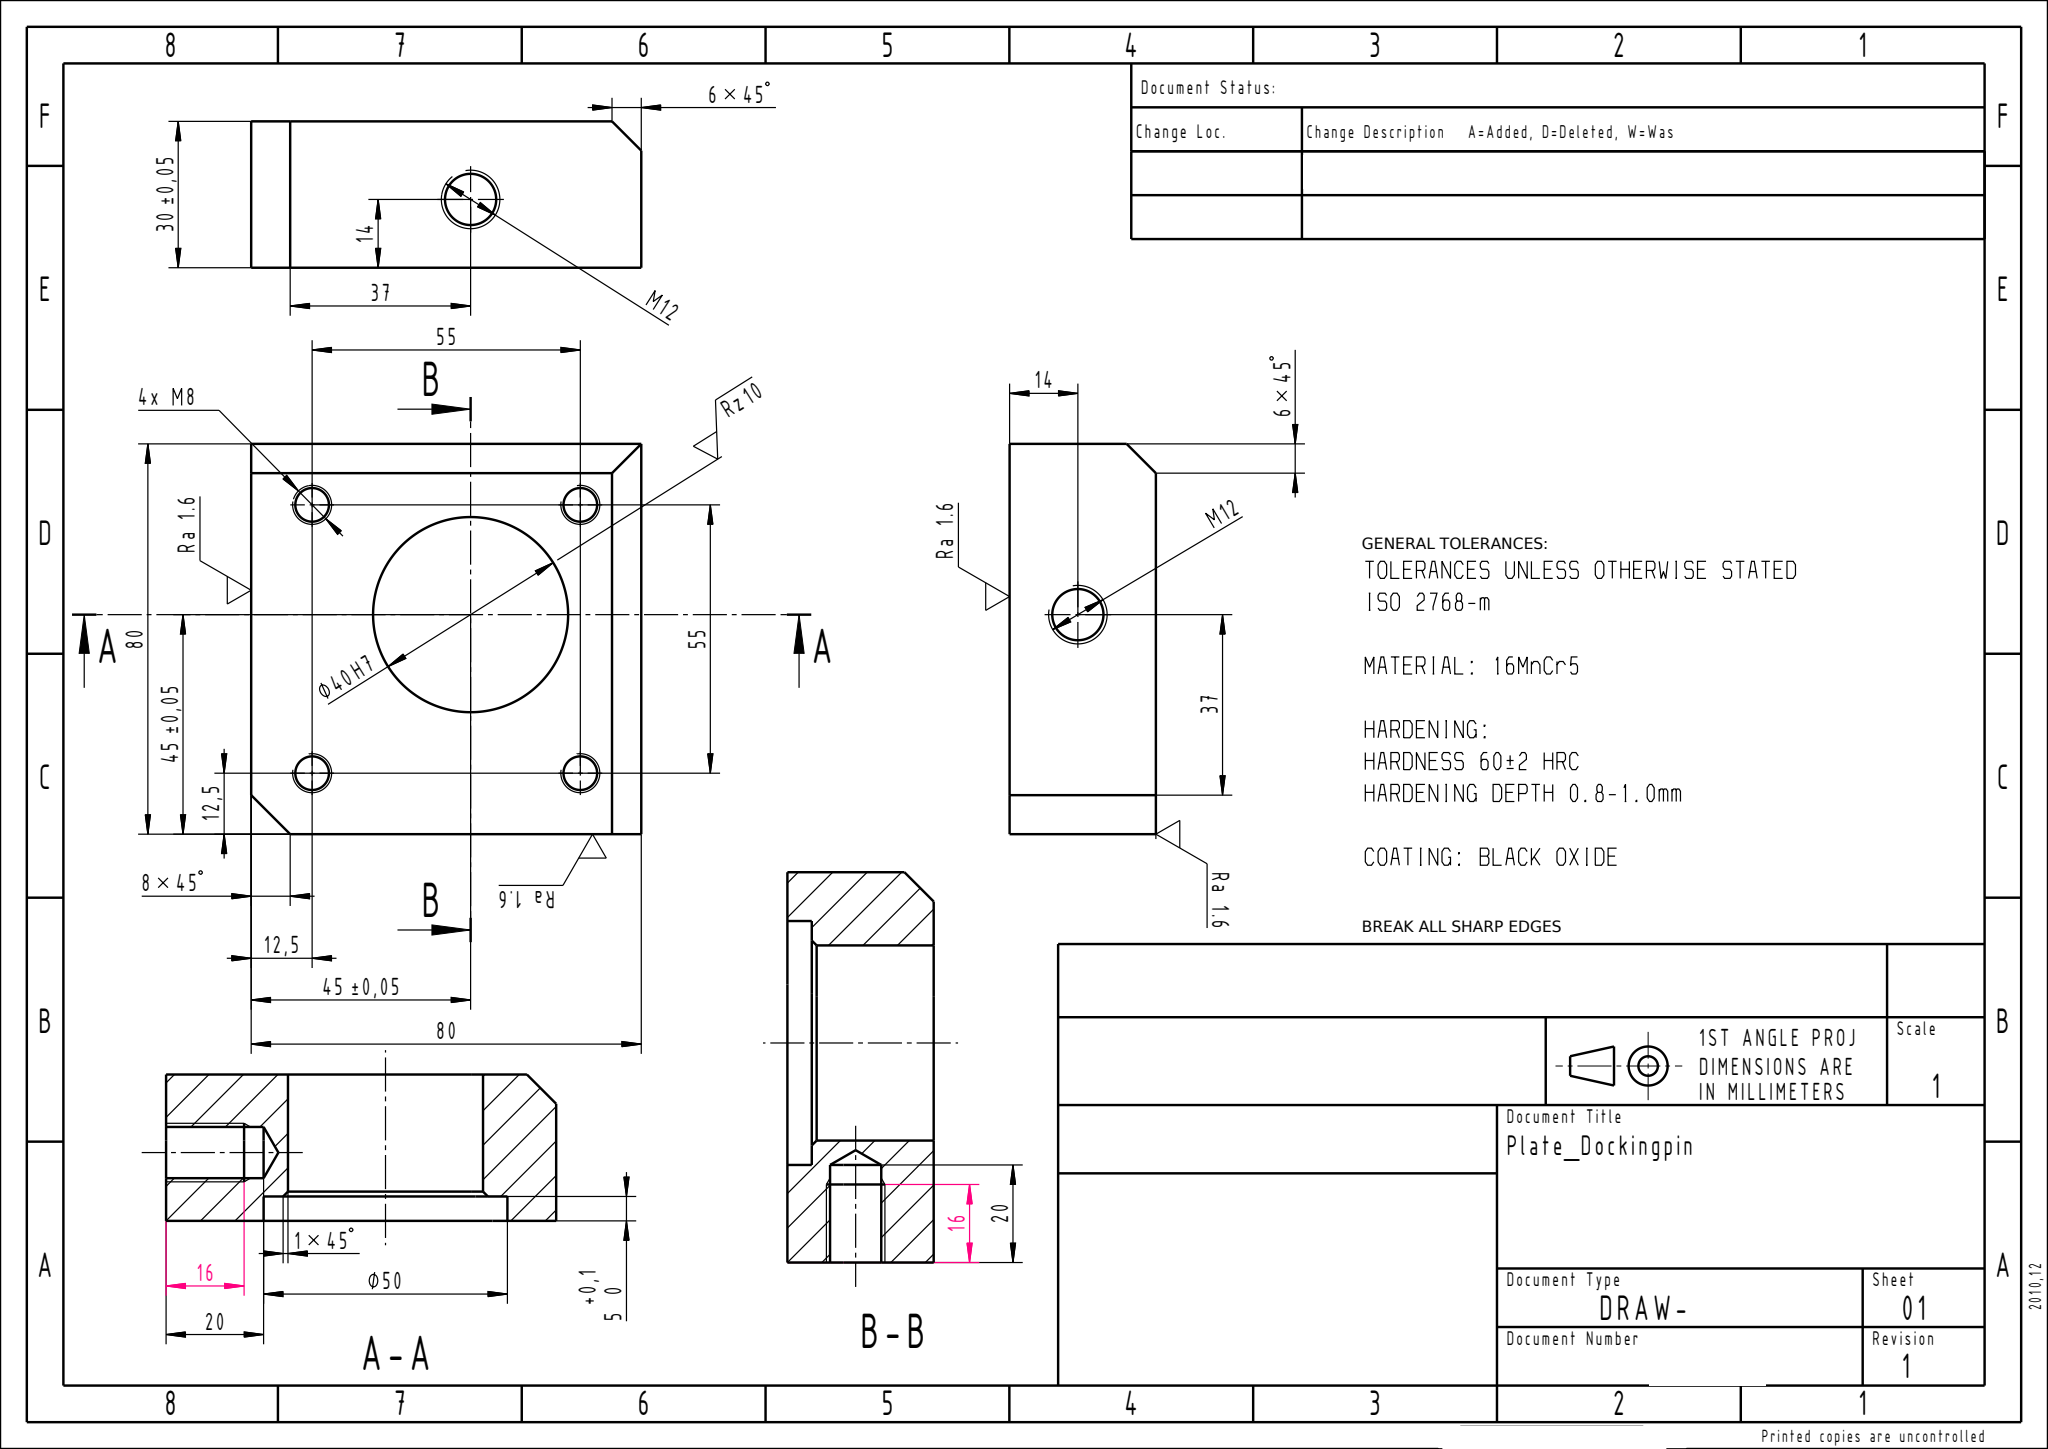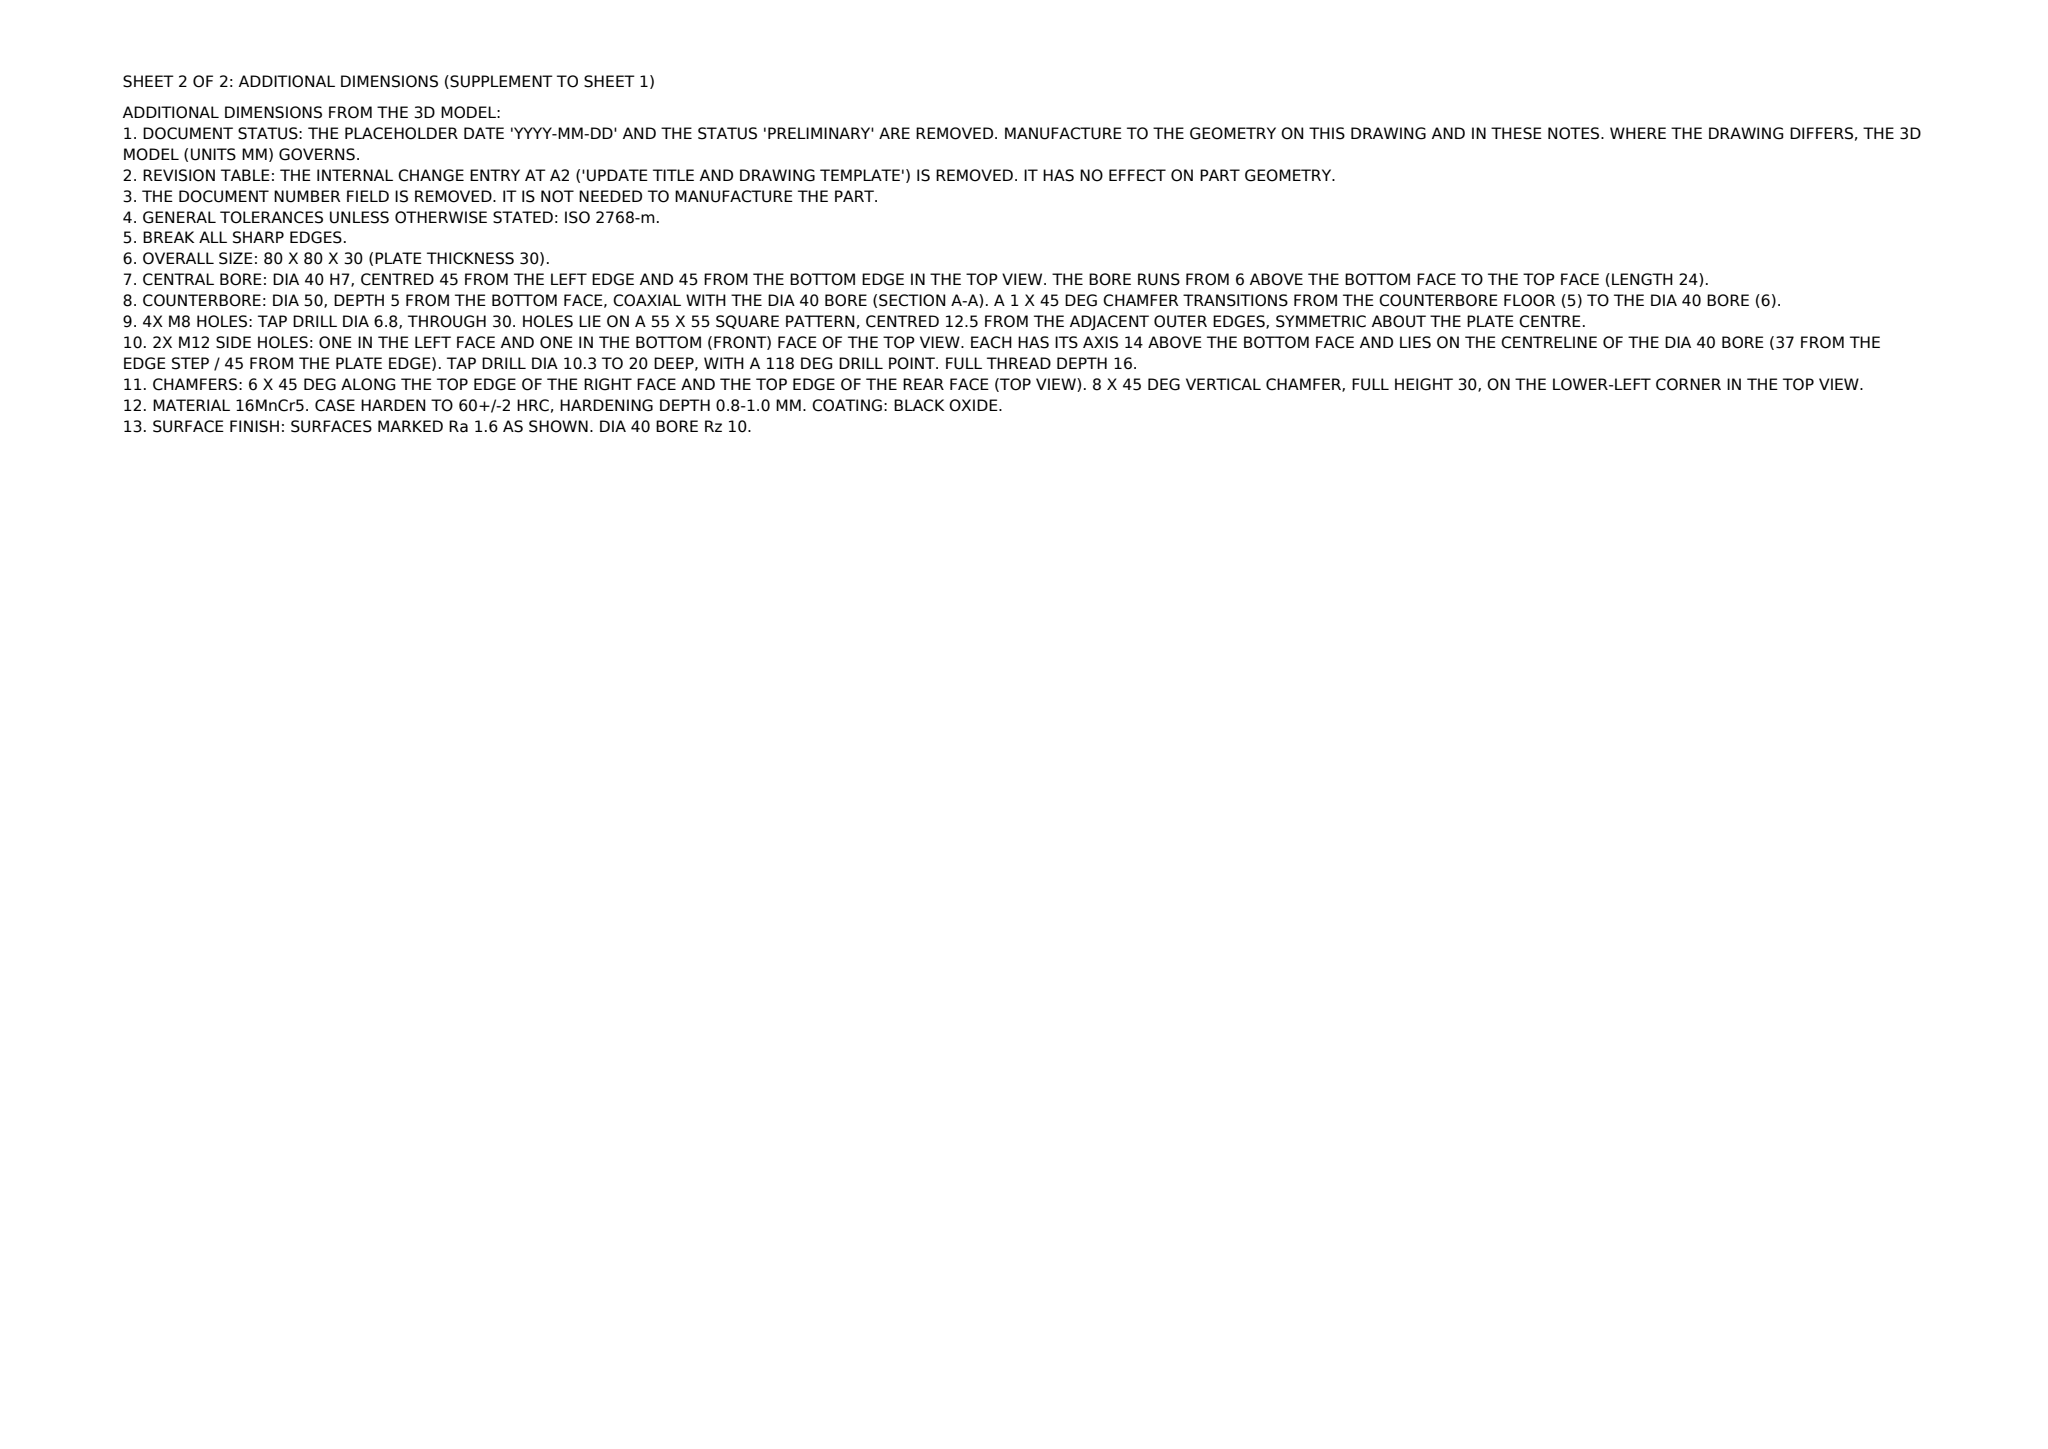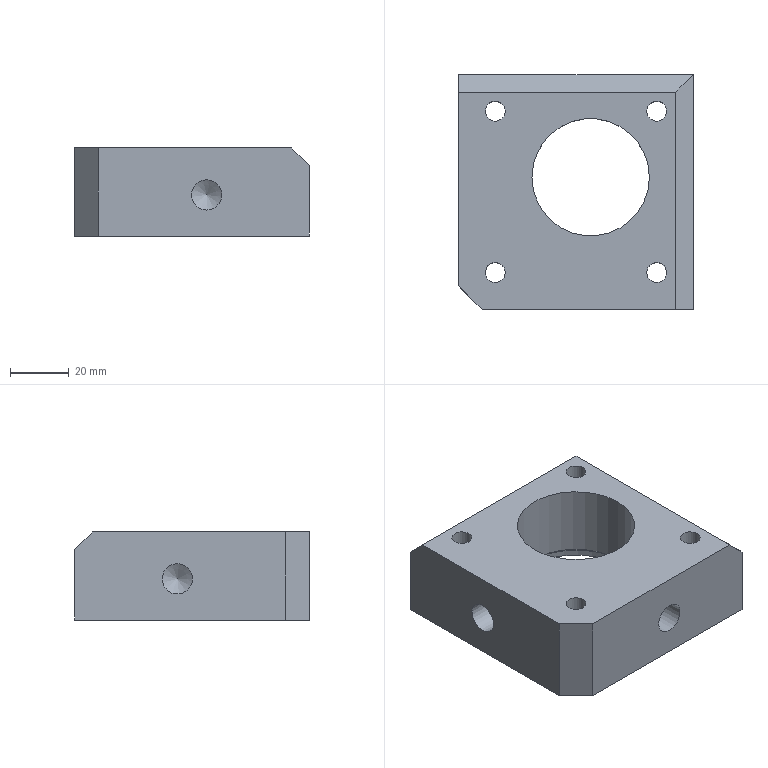Part | NX | mm | 1 solid | 21 faces | box 80 x 80 x 30 mm | volume 139072 mm3 | plane 10 | cylinder 8 | cone 3 | commonest cylinder face diameters 6.8 x4 10.3 x2 40 x1 50 x1
STEP:
#1=CARTESIAN_POINT('',(0.,0.,0.));
#2=DIRECTION('',(0.,0.,1.));
#3=DIRECTION('',(1.,0.,0.));
#4=AXIS2_PLACEMENT_3D('',#1,#2,#3);
#5=(LENGTH_UNIT()NAMED_UNIT(*)SI_UNIT(.MILLI.,.METRE.));
#6=UNCERTAINTY_MEASURE_WITH_UNIT(LENGTH_MEASURE(0.00002),#5,'','');
#7=(NAMED_UNIT(*)PLANE_ANGLE_UNIT()SI_UNIT($,.RADIAN.));
#8=PLANE_ANGLE_MEASURE_WITH_UNIT(PLANE_ANGLE_MEASURE(0.01745),#7);
#9=DIMENSIONAL_EXPONENTS(0.,0.,0.,0.,0.,0.,0.);
#10=(CONVERSION_BASED_UNIT('',#8)NAMED_UNIT(#9)PLANE_ANGLE_UNIT());
#11=(NAMED_UNIT(*)SI_UNIT($,.STERADIAN.)SOLID_ANGLE_UNIT());
#12=(GEOMETRIC_REPRESENTATION_CONTEXT(3)GLOBAL_UNCERTAINTY_ASSIGNED_CONTEXT((#6))GLOBAL_UNIT_ASSIGNED_CONTEXT((#5,#10,#11))REPRESENTATION_CONTEXT('',''));
#13=SHAPE_REPRESENTATION('',(#4),#12);
#14=CARTESIAN_POINT('',(-40.,10.15,14.));
#15=VERTEX_POINT('',#14);
#16=CARTESIAN_POINT('',(-40.,5.,14.));
#17=DIRECTION('',(1.,0.,0.));
#18=DIRECTION('',(-0.,1.,0.));
#19=AXIS2_PLACEMENT_3D('',#16,#17,#18);
#20=CIRCLE('',#19,5.15);
#21=EDGE_CURVE('',#15,#15,#20,.T.);
#22=ORIENTED_EDGE('',*,*,#21,.T.);
#23=EDGE_LOOP('',(#22));
#24=FACE_BOUND('',#23,.T.);
#25=CARTESIAN_POINT('',(-40.,34.,30.));
#26=VERTEX_POINT('',#25);
#27=CARTESIAN_POINT('',(-40.,-32.,30.));
#28=VERTEX_POINT('',#27);
#29=CARTESIAN_POINT('',(-40.,40.,30.));
#30=DIRECTION('',(0.,-1.,0.));
#31=VECTOR('',#30,1.);
#32=LINE('',#29,#31);
#33=EDGE_CURVE('',#26,#28,#32,.T.);
#34=ORIENTED_EDGE('',*,*,#33,.F.);
#35=CARTESIAN_POINT('',(-40.,40.,24.));
#36=VERTEX_POINT('',#35);
#37=CARTESIAN_POINT('',(-40.,34.,30.));
#38=DIRECTION('',(-0.,0.7071,-0.7071));
#39=VECTOR('',#38,1.);
#40=LINE('',#37,#39);
#41=EDGE_CURVE('',#26,#36,#40,.T.);
#42=ORIENTED_EDGE('',*,*,#41,.T.);
#43=CARTESIAN_POINT('',(-40.,40.,0.));
#44=VERTEX_POINT('',#43);
#45=CARTESIAN_POINT('',(-40.,40.,30.));
#46=DIRECTION('',(0.,0.,-1.));
#47=VECTOR('',#46,1.);
#48=LINE('',#45,#47);
#49=EDGE_CURVE('',#36,#44,#48,.T.);
#50=ORIENTED_EDGE('',*,*,#49,.T.);
#51=CARTESIAN_POINT('',(-40.,-32.,0.));
#52=VERTEX_POINT('',#51);
#53=CARTESIAN_POINT('',(-40.,40.,0.));
#54=DIRECTION('',(0.,-1.,0.));
#55=VECTOR('',#54,1.);
#56=LINE('',#53,#55);
#57=EDGE_CURVE('',#44,#52,#56,.T.);
#58=ORIENTED_EDGE('',*,*,#57,.T.);
#59=CARTESIAN_POINT('',(-40.,-32.,30.));
#60=DIRECTION('',(0.,0.,1.));
#61=VECTOR('',#60,1.);
#62=LINE('',#59,#61);
#63=EDGE_CURVE('',#52,#28,#62,.T.);
#64=ORIENTED_EDGE('',*,*,#63,.T.);
#65=EDGE_LOOP('',(#34,#42,#50,#58,#64));
#66=FACE_BOUND('',#65,.T.);
#67=CARTESIAN_POINT('',(-40.,40.,30.));
#68=DIRECTION('',(1.,0.,0.));
#69=DIRECTION('',(-0.,1.,0.));
#70=AXIS2_PLACEMENT_3D('',#67,#68,#69);
#71=PLANE('',#70);
#72=ADVANCED_FACE('',(#24,#66),#71,.F.);
#73=CARTESIAN_POINT('',(5.,-40.,19.15));
#74=VERTEX_POINT('',#73);
#75=CARTESIAN_POINT('',(5.,-40.,14.));
#76=DIRECTION('',(0.,1.,0.));
#77=DIRECTION('',(0.,0.,1.));
#78=AXIS2_PLACEMENT_3D('',#75,#76,#77);
#79=CIRCLE('',#78,5.15);
#80=EDGE_CURVE('',#74,#74,#79,.T.);
#81=ORIENTED_EDGE('',*,*,#80,.T.);
#82=EDGE_LOOP('',(#81));
#83=FACE_BOUND('',#82,.T.);
#84=CARTESIAN_POINT('',(40.,-40.,24.));
#85=VERTEX_POINT('',#84);
#86=CARTESIAN_POINT('',(40.,-40.,0.));
#87=VERTEX_POINT('',#86);
#88=CARTESIAN_POINT('',(40.,-40.,30.));
#89=DIRECTION('',(0.,0.,-1.));
#90=VECTOR('',#89,1.);
#91=LINE('',#88,#90);
#92=EDGE_CURVE('',#85,#87,#91,.T.);
#93=ORIENTED_EDGE('',*,*,#92,.F.);
#94=CARTESIAN_POINT('',(34.,-40.,30.));
#95=VERTEX_POINT('',#94);
#96=CARTESIAN_POINT('',(34.,-40.,30.));
#97=DIRECTION('',(-0.7071,0.,0.7071));
#98=VECTOR('',#97,1.);
#99=LINE('',#96,#98);
#100=EDGE_CURVE('',#85,#95,#99,.T.);
#101=ORIENTED_EDGE('',*,*,#100,.T.);
#102=CARTESIAN_POINT('',(-32.,-40.,30.));
#103=VERTEX_POINT('',#102);
#104=CARTESIAN_POINT('',(-40.,-40.,30.));
#105=DIRECTION('',(1.,0.,0.));
#106=VECTOR('',#105,1.);
#107=LINE('',#104,#106);
#108=EDGE_CURVE('',#103,#95,#107,.T.);
#109=ORIENTED_EDGE('',*,*,#108,.F.);
#110=CARTESIAN_POINT('',(-32.,-40.,0.));
#111=VERTEX_POINT('',#110);
#112=CARTESIAN_POINT('',(-32.,-40.,30.));
#113=DIRECTION('',(0.,0.,-1.));
#114=VECTOR('',#113,1.);
#115=LINE('',#112,#114);
#116=EDGE_CURVE('',#103,#111,#115,.T.);
#117=ORIENTED_EDGE('',*,*,#116,.T.);
#118=CARTESIAN_POINT('',(-40.,-40.,0.));
#119=DIRECTION('',(1.,0.,0.));
#120=VECTOR('',#119,1.);
#121=LINE('',#118,#120);
#122=EDGE_CURVE('',#111,#87,#121,.T.);
#123=ORIENTED_EDGE('',*,*,#122,.T.);
#124=EDGE_LOOP('',(#93,#101,#109,#117,#123));
#125=FACE_BOUND('',#124,.T.);
#126=CARTESIAN_POINT('',(-40.,-40.,30.));
#127=DIRECTION('',(0.,1.,0.));
#128=DIRECTION('',(0.,0.,1.));
#129=AXIS2_PLACEMENT_3D('',#126,#127,#128);
#130=PLANE('',#129);
#131=ADVANCED_FACE('',(#83,#125),#130,.F.);
#132=CARTESIAN_POINT('',(40.,40.,24.));
#133=VERTEX_POINT('',#132);
#134=CARTESIAN_POINT('',(40.,40.,0.));
#135=VERTEX_POINT('',#134);
#136=CARTESIAN_POINT('',(40.,40.,30.));
#137=DIRECTION('',(0.,0.,-1.));
#138=VECTOR('',#137,1.);
#139=LINE('',#136,#138);
#140=EDGE_CURVE('',#133,#135,#139,.T.);
#141=ORIENTED_EDGE('',*,*,#140,.F.);
#142=CARTESIAN_POINT('',(40.,-40.,24.));
#143=DIRECTION('',(0.,-1.,0.));
#144=VECTOR('',#143,1.);
#145=LINE('',#142,#144);
#146=EDGE_CURVE('',#133,#85,#145,.T.);
#147=ORIENTED_EDGE('',*,*,#146,.T.);
#148=ORIENTED_EDGE('',*,*,#92,.T.);
#149=CARTESIAN_POINT('',(40.,-40.,0.));
#150=DIRECTION('',(-0.,1.,0.));
#151=VECTOR('',#150,1.);
#152=LINE('',#149,#151);
#153=EDGE_CURVE('',#87,#135,#152,.T.);
#154=ORIENTED_EDGE('',*,*,#153,.T.);
#155=EDGE_LOOP('',(#141,#147,#148,#154));
#156=FACE_OUTER_BOUND('',#155,.T.);
#157=CARTESIAN_POINT('',(40.,-40.,30.));
#158=DIRECTION('',(-1.,-0.,0.));
#159=DIRECTION('',(0.,-1.,0.));
#160=AXIS2_PLACEMENT_3D('',#157,#158,#159);
#161=PLANE('',#160);
#162=ADVANCED_FACE('',(#156),#161,.F.);
#163=ORIENTED_EDGE('',*,*,#49,.F.);
#164=CARTESIAN_POINT('',(40.,40.,24.));
#165=DIRECTION('',(1.,0.,0.));
#166=VECTOR('',#165,1.);
#167=LINE('',#164,#166);
#168=EDGE_CURVE('',#36,#133,#167,.T.);
#169=ORIENTED_EDGE('',*,*,#168,.T.);
#170=ORIENTED_EDGE('',*,*,#140,.T.);
#171=CARTESIAN_POINT('',(40.,40.,0.));
#172=DIRECTION('',(-1.,0.,0.));
#173=VECTOR('',#172,1.);
#174=LINE('',#171,#173);
#175=EDGE_CURVE('',#135,#44,#174,.T.);
#176=ORIENTED_EDGE('',*,*,#175,.T.);
#177=EDGE_LOOP('',(#163,#169,#170,#176));
#178=FACE_OUTER_BOUND('',#177,.T.);
#179=CARTESIAN_POINT('',(40.,40.,30.));
#180=DIRECTION('',(0.,-1.,0.));
#181=DIRECTION('',(0.,0.,-1.));
#182=AXIS2_PLACEMENT_3D('',#179,#180,#181);
#183=PLANE('',#182);
#184=ADVANCED_FACE('',(#178),#183,.F.);
#185=CARTESIAN_POINT('',(30.9,27.5,30.));
#186=VERTEX_POINT('',#185);
#187=CARTESIAN_POINT('',(27.5,27.5,30.));
#188=DIRECTION('',(0.,0.,1.));
#189=DIRECTION('',(1.,0.,0.));
#190=AXIS2_PLACEMENT_3D('',#187,#188,#189);
#191=CIRCLE('',#190,3.4);
#192=EDGE_CURVE('',#186,#186,#191,.T.);
#193=ORIENTED_EDGE('',*,*,#192,.F.);
#194=EDGE_LOOP('',(#193));
#195=FACE_BOUND('',#194,.T.);
#196=CARTESIAN_POINT('',(30.9,-27.5,30.));
#197=VERTEX_POINT('',#196);
#198=CARTESIAN_POINT('',(27.5,-27.5,30.));
#199=DIRECTION('',(0.,0.,1.));
#200=DIRECTION('',(1.,0.,0.));
#201=AXIS2_PLACEMENT_3D('',#198,#199,#200);
#202=CIRCLE('',#201,3.4);
#203=EDGE_CURVE('',#197,#197,#202,.T.);
#204=ORIENTED_EDGE('',*,*,#203,.F.);
#205=EDGE_LOOP('',(#204));
#206=FACE_BOUND('',#205,.T.);
#207=CARTESIAN_POINT('',(-24.1,27.5,30.));
#208=VERTEX_POINT('',#207);
#209=CARTESIAN_POINT('',(-27.5,27.5,30.));
#210=DIRECTION('',(0.,0.,1.));
#211=DIRECTION('',(1.,0.,0.));
#212=AXIS2_PLACEMENT_3D('',#209,#210,#211);
#213=CIRCLE('',#212,3.4);
#214=EDGE_CURVE('',#208,#208,#213,.T.);
#215=ORIENTED_EDGE('',*,*,#214,.F.);
#216=EDGE_LOOP('',(#215));
#217=FACE_BOUND('',#216,.T.);
#218=CARTESIAN_POINT('',(-24.1,-27.5,30.));
#219=VERTEX_POINT('',#218);
#220=CARTESIAN_POINT('',(-27.5,-27.5,30.));
#221=DIRECTION('',(0.,0.,1.));
#222=DIRECTION('',(1.,0.,0.));
#223=AXIS2_PLACEMENT_3D('',#220,#221,#222);
#224=CIRCLE('',#223,3.4);
#225=EDGE_CURVE('',#219,#219,#224,.T.);
#226=ORIENTED_EDGE('',*,*,#225,.F.);
#227=EDGE_LOOP('',(#226));
#228=FACE_BOUND('',#227,.T.);
#229=CARTESIAN_POINT('',(25.,5.,30.));
#230=VERTEX_POINT('',#229);
#231=CARTESIAN_POINT('',(5.,5.,30.));
#232=DIRECTION('',(0.,0.,1.));
#233=DIRECTION('',(1.,0.,0.));
#234=AXIS2_PLACEMENT_3D('',#231,#232,#233);
#235=CIRCLE('',#234,20.);
#236=EDGE_CURVE('',#230,#230,#235,.T.);
#237=ORIENTED_EDGE('',*,*,#236,.F.);
#238=EDGE_LOOP('',(#237));
#239=FACE_BOUND('',#238,.T.);
#240=CARTESIAN_POINT('',(34.,34.,30.));
#241=VERTEX_POINT('',#240);
#242=CARTESIAN_POINT('',(34.,40.,30.));
#243=DIRECTION('',(-0.,1.,0.));
#244=VECTOR('',#243,1.);
#245=LINE('',#242,#244);
#246=EDGE_CURVE('',#95,#241,#245,.T.);
#247=ORIENTED_EDGE('',*,*,#246,.T.);
#248=CARTESIAN_POINT('',(-40.,34.,30.));
#249=DIRECTION('',(-1.,0.,0.));
#250=VECTOR('',#249,1.);
#251=LINE('',#248,#250);
#252=EDGE_CURVE('',#241,#26,#251,.T.);
#253=ORIENTED_EDGE('',*,*,#252,.T.);
#254=ORIENTED_EDGE('',*,*,#33,.T.);
#255=CARTESIAN_POINT('',(-36.,-36.,30.));
#256=DIRECTION('',(0.7071,-0.7071,0.));
#257=VECTOR('',#256,1.);
#258=LINE('',#255,#257);
#259=EDGE_CURVE('',#28,#103,#258,.T.);
#260=ORIENTED_EDGE('',*,*,#259,.T.);
#261=ORIENTED_EDGE('',*,*,#108,.T.);
#262=EDGE_LOOP('',(#247,#253,#254,#260,#261));
#263=FACE_BOUND('',#262,.T.);
#264=CARTESIAN_POINT('',(0.,0.,30.));
#265=DIRECTION('',(0.,0.,1.));
#266=DIRECTION('',(1.,0.,0.));
#267=AXIS2_PLACEMENT_3D('',#264,#265,#266);
#268=PLANE('',#267);
#269=ADVANCED_FACE('',(#195,#206,#217,#228,#239,#263),#268,.T.);
#270=CARTESIAN_POINT('',(30.9,27.5,0.));
#271=VERTEX_POINT('',#270);
#272=CARTESIAN_POINT('',(27.5,27.5,0.));
#273=DIRECTION('',(0.,0.,1.));
#274=DIRECTION('',(1.,0.,0.));
#275=AXIS2_PLACEMENT_3D('',#272,#273,#274);
#276=CIRCLE('',#275,3.4);
#277=EDGE_CURVE('',#271,#271,#276,.T.);
#278=ORIENTED_EDGE('',*,*,#277,.T.);
#279=EDGE_LOOP('',(#278));
#280=FACE_BOUND('',#279,.T.);
#281=CARTESIAN_POINT('',(30.9,-27.5,0.));
#282=VERTEX_POINT('',#281);
#283=CARTESIAN_POINT('',(27.5,-27.5,0.));
#284=DIRECTION('',(0.,0.,1.));
#285=DIRECTION('',(1.,0.,0.));
#286=AXIS2_PLACEMENT_3D('',#283,#284,#285);
#287=CIRCLE('',#286,3.4);
#288=EDGE_CURVE('',#282,#282,#287,.T.);
#289=ORIENTED_EDGE('',*,*,#288,.T.);
#290=EDGE_LOOP('',(#289));
#291=FACE_BOUND('',#290,.T.);
#292=CARTESIAN_POINT('',(-24.1,27.5,0.));
#293=VERTEX_POINT('',#292);
#294=CARTESIAN_POINT('',(-27.5,27.5,0.));
#295=DIRECTION('',(0.,0.,1.));
#296=DIRECTION('',(1.,0.,0.));
#297=AXIS2_PLACEMENT_3D('',#294,#295,#296);
#298=CIRCLE('',#297,3.4);
#299=EDGE_CURVE('',#293,#293,#298,.T.);
#300=ORIENTED_EDGE('',*,*,#299,.T.);
#301=EDGE_LOOP('',(#300));
#302=FACE_BOUND('',#301,.T.);
#303=CARTESIAN_POINT('',(-24.1,-27.5,0.));
#304=VERTEX_POINT('',#303);
#305=CARTESIAN_POINT('',(-27.5,-27.5,0.));
#306=DIRECTION('',(0.,0.,1.));
#307=DIRECTION('',(1.,0.,0.));
#308=AXIS2_PLACEMENT_3D('',#305,#306,#307);
#309=CIRCLE('',#308,3.4);
#310=EDGE_CURVE('',#304,#304,#309,.T.);
#311=ORIENTED_EDGE('',*,*,#310,.T.);
#312=EDGE_LOOP('',(#311));
#313=FACE_BOUND('',#312,.T.);
#314=CARTESIAN_POINT('',(30.,5.,0.));
#315=VERTEX_POINT('',#314);
#316=CARTESIAN_POINT('',(5.,5.,0.));
#317=DIRECTION('',(0.,0.,1.));
#318=DIRECTION('',(1.,0.,0.));
#319=AXIS2_PLACEMENT_3D('',#316,#317,#318);
#320=CIRCLE('',#319,25.);
#321=EDGE_CURVE('',#315,#315,#320,.T.);
#322=ORIENTED_EDGE('',*,*,#321,.T.);
#323=EDGE_LOOP('',(#322));
#324=FACE_BOUND('',#323,.T.);
#325=ORIENTED_EDGE('',*,*,#122,.F.);
#326=CARTESIAN_POINT('',(-32.,-40.,0.));
#327=DIRECTION('',(-0.7071,0.7071,0.));
#328=VECTOR('',#327,1.);
#329=LINE('',#326,#328);
#330=EDGE_CURVE('',#111,#52,#329,.T.);
#331=ORIENTED_EDGE('',*,*,#330,.T.);
#332=ORIENTED_EDGE('',*,*,#57,.F.);
#333=ORIENTED_EDGE('',*,*,#175,.F.);
#334=ORIENTED_EDGE('',*,*,#153,.F.);
#335=EDGE_LOOP('',(#325,#331,#332,#333,#334));
#336=FACE_BOUND('',#335,.T.);
#337=CARTESIAN_POINT('',(0.,0.,0.));
#338=DIRECTION('',(0.,0.,1.));
#339=DIRECTION('',(1.,0.,0.));
#340=AXIS2_PLACEMENT_3D('',#337,#338,#339);
#341=PLANE('',#340);
#342=ADVANCED_FACE('',(#280,#291,#302,#313,#324,#336),#341,.F.);
#343=ORIENTED_EDGE('',*,*,#100,.F.);
#344=ORIENTED_EDGE('',*,*,#146,.F.);
#345=CARTESIAN_POINT('',(22.667,22.667,41.333));
#346=DIRECTION('',(0.5774,0.5774,-0.5774));
#347=VECTOR('',#346,1.);
#348=LINE('',#345,#347);
#349=EDGE_CURVE('',#241,#133,#348,.T.);
#350=ORIENTED_EDGE('',*,*,#349,.F.);
#351=ORIENTED_EDGE('',*,*,#246,.F.);
#352=EDGE_LOOP('',(#343,#344,#350,#351));
#353=FACE_OUTER_BOUND('',#352,.T.);
#354=CARTESIAN_POINT('',(34.,0.,30.));
#355=DIRECTION('',(0.7071,0.,0.7071));
#356=DIRECTION('',(0.,-1.,0.));
#357=AXIS2_PLACEMENT_3D('',#354,#355,#356);
#358=PLANE('',#357);
#359=ADVANCED_FACE('',(#353),#358,.T.);
#360=ORIENTED_EDGE('',*,*,#349,.T.);
#361=ORIENTED_EDGE('',*,*,#168,.F.);
#362=ORIENTED_EDGE('',*,*,#41,.F.);
#363=ORIENTED_EDGE('',*,*,#252,.F.);
#364=EDGE_LOOP('',(#360,#361,#362,#363));
#365=FACE_OUTER_BOUND('',#364,.T.);
#366=CARTESIAN_POINT('',(0.,34.,30.));
#367=DIRECTION('',(0.,0.7071,0.7071));
#368=DIRECTION('',(1.,0.,0.));
#369=AXIS2_PLACEMENT_3D('',#366,#367,#368);
#370=PLANE('',#369);
#371=ADVANCED_FACE('',(#365),#370,.T.);
#372=ORIENTED_EDGE('',*,*,#259,.F.);
#373=ORIENTED_EDGE('',*,*,#63,.F.);
#374=ORIENTED_EDGE('',*,*,#330,.F.);
#375=ORIENTED_EDGE('',*,*,#116,.F.);
#376=EDGE_LOOP('',(#372,#373,#374,#375));
#377=FACE_OUTER_BOUND('',#376,.T.);
#378=CARTESIAN_POINT('',(-32.,-40.,30.));
#379=DIRECTION('',(0.7071,0.7071,0.));
#380=DIRECTION('',(0.,0.,-1.));
#381=AXIS2_PLACEMENT_3D('',#378,#379,#380);
#382=PLANE('',#381);
#383=ADVANCED_FACE('',(#377),#382,.F.);
#384=ORIENTED_EDGE('',*,*,#236,.T.);
#385=EDGE_LOOP('',(#384));
#386=FACE_BOUND('',#385,.T.);
#387=CARTESIAN_POINT('',(25.,5.,6.));
#388=VERTEX_POINT('',#387);
#389=CARTESIAN_POINT('',(5.,5.,6.));
#390=DIRECTION('',(0.,0.,-1.));
#391=DIRECTION('',(1.,0.,0.));
#392=AXIS2_PLACEMENT_3D('',#389,#390,#391);
#393=CIRCLE('',#392,20.);
#394=EDGE_CURVE('',#388,#388,#393,.T.);
#395=ORIENTED_EDGE('',*,*,#394,.T.);
#396=EDGE_LOOP('',(#395));
#397=FACE_BOUND('',#396,.T.);
#398=CARTESIAN_POINT('',(5.,5.,78.986));
#399=DIRECTION('',(0.,0.,1.));
#400=DIRECTION('',(1.,0.,0.));
#401=AXIS2_PLACEMENT_3D('',#398,#399,#400);
#402=CYLINDRICAL_SURFACE('',#401,20.);
#403=ADVANCED_FACE('',(#386,#397),#402,.F.);
#404=CARTESIAN_POINT('',(26.,5.,5.));
#405=VERTEX_POINT('',#404);
#406=CARTESIAN_POINT('',(5.,5.,5.));
#407=DIRECTION('',(0.,0.,1.));
#408=DIRECTION('',(1.,0.,0.));
#409=AXIS2_PLACEMENT_3D('',#406,#407,#408);
#410=CIRCLE('',#409,21.);
#411=EDGE_CURVE('',#405,#405,#410,.T.);
#412=ORIENTED_EDGE('',*,*,#411,.T.);
#413=EDGE_LOOP('',(#412));
#414=FACE_BOUND('',#413,.T.);
#415=CARTESIAN_POINT('',(30.,5.,5.));
#416=VERTEX_POINT('',#415);
#417=CARTESIAN_POINT('',(5.,5.,5.));
#418=DIRECTION('',(0.,0.,-1.));
#419=DIRECTION('',(1.,0.,0.));
#420=AXIS2_PLACEMENT_3D('',#417,#418,#419);
#421=CIRCLE('',#420,25.);
#422=EDGE_CURVE('',#416,#416,#421,.T.);
#423=ORIENTED_EDGE('',*,*,#422,.T.);
#424=EDGE_LOOP('',(#423));
#425=FACE_BOUND('',#424,.T.);
#426=CARTESIAN_POINT('',(5.,5.,5.));
#427=DIRECTION('',(0.,0.,1.));
#428=DIRECTION('',(1.,0.,0.));
#429=AXIS2_PLACEMENT_3D('',#426,#427,#428);
#430=PLANE('',#429);
#431=ADVANCED_FACE('',(#414,#425),#430,.F.);
#432=ORIENTED_EDGE('',*,*,#422,.F.);
#433=EDGE_LOOP('',(#432));
#434=FACE_BOUND('',#433,.T.);
#435=ORIENTED_EDGE('',*,*,#321,.F.);
#436=EDGE_LOOP('',(#435));
#437=FACE_BOUND('',#436,.T.);
#438=CARTESIAN_POINT('',(5.,5.,0.));
#439=DIRECTION('',(0.,0.,1.));
#440=DIRECTION('',(1.,0.,0.));
#441=AXIS2_PLACEMENT_3D('',#438,#439,#440);
#442=CYLINDRICAL_SURFACE('',#441,25.);
#443=ADVANCED_FACE('',(#434,#437),#442,.F.);
#444=ORIENTED_EDGE('',*,*,#411,.F.);
#445=EDGE_LOOP('',(#444));
#446=FACE_BOUND('',#445,.T.);
#447=ORIENTED_EDGE('',*,*,#394,.F.);
#448=EDGE_LOOP('',(#447));
#449=FACE_BOUND('',#448,.T.);
#450=CARTESIAN_POINT('',(5.,5.,6.));
#451=DIRECTION('',(0.,0.,-1.));
#452=DIRECTION('',(-1.,0.,0.));
#453=AXIS2_PLACEMENT_3D('',#450,#451,#452);
#454=CONICAL_SURFACE('',#453,20.,45.);
#455=ADVANCED_FACE('',(#446,#449),#454,.F.);
#456=CARTESIAN_POINT('',(-20.,10.15,14.));
#457=VERTEX_POINT('',#456);
#458=CARTESIAN_POINT('',(-20.,5.,14.));
#459=DIRECTION('',(-1.,-0.,0.));
#460=DIRECTION('',(-0.,1.,0.));
#461=AXIS2_PLACEMENT_3D('',#458,#459,#460);
#462=CIRCLE('',#461,5.15);
#463=EDGE_CURVE('',#457,#457,#462,.T.);
#464=ORIENTED_EDGE('',*,*,#463,.T.);
#465=EDGE_LOOP('',(#464));
#466=FACE_BOUND('',#465,.T.);
#467=CARTESIAN_POINT('',(-16.906,5.,14.));
#468=VERTEX_POINT('',#467);
#469=VERTEX_LOOP('',#468);
#470=FACE_BOUND('',#469,.T.);
#471=CARTESIAN_POINT('',(-20.,5.,14.));
#472=DIRECTION('',(-1.,-0.,0.));
#473=DIRECTION('',(0.,-1.,0.));
#474=AXIS2_PLACEMENT_3D('',#471,#472,#473);
#475=CONICAL_SURFACE('',#474,5.15,59.);
#476=ADVANCED_FACE('',(#466,#470),#475,.F.);
#477=ORIENTED_EDGE('',*,*,#463,.F.);
#478=EDGE_LOOP('',(#477));
#479=FACE_BOUND('',#478,.T.);
#480=ORIENTED_EDGE('',*,*,#21,.F.);
#481=EDGE_LOOP('',(#480));
#482=FACE_BOUND('',#481,.T.);
#483=CARTESIAN_POINT('',(-40.,5.,14.));
#484=DIRECTION('',(1.,0.,0.));
#485=DIRECTION('',(-0.,1.,0.));
#486=AXIS2_PLACEMENT_3D('',#483,#484,#485);
#487=CYLINDRICAL_SURFACE('',#486,5.15);
#488=ADVANCED_FACE('',(#479,#482),#487,.F.);
#489=ORIENTED_EDGE('',*,*,#225,.T.);
#490=EDGE_LOOP('',(#489));
#491=FACE_BOUND('',#490,.T.);
#492=ORIENTED_EDGE('',*,*,#310,.F.);
#493=EDGE_LOOP('',(#492));
#494=FACE_BOUND('',#493,.T.);
#495=CARTESIAN_POINT('',(-27.5,-27.5,0.));
#496=DIRECTION('',(0.,0.,1.));
#497=DIRECTION('',(1.,0.,0.));
#498=AXIS2_PLACEMENT_3D('',#495,#496,#497);
#499=CYLINDRICAL_SURFACE('',#498,3.4);
#500=ADVANCED_FACE('',(#491,#494),#499,.F.);
#501=ORIENTED_EDGE('',*,*,#214,.T.);
#502=EDGE_LOOP('',(#501));
#503=FACE_BOUND('',#502,.T.);
#504=ORIENTED_EDGE('',*,*,#299,.F.);
#505=EDGE_LOOP('',(#504));
#506=FACE_BOUND('',#505,.T.);
#507=CARTESIAN_POINT('',(-27.5,27.5,0.));
#508=DIRECTION('',(0.,0.,1.));
#509=DIRECTION('',(1.,0.,0.));
#510=AXIS2_PLACEMENT_3D('',#507,#508,#509);
#511=CYLINDRICAL_SURFACE('',#510,3.4);
#512=ADVANCED_FACE('',(#503,#506),#511,.F.);
#513=ORIENTED_EDGE('',*,*,#203,.T.);
#514=EDGE_LOOP('',(#513));
#515=FACE_BOUND('',#514,.T.);
#516=ORIENTED_EDGE('',*,*,#288,.F.);
#517=EDGE_LOOP('',(#516));
#518=FACE_BOUND('',#517,.T.);
#519=CARTESIAN_POINT('',(27.5,-27.5,0.));
#520=DIRECTION('',(0.,0.,1.));
#521=DIRECTION('',(1.,0.,0.));
#522=AXIS2_PLACEMENT_3D('',#519,#520,#521);
#523=CYLINDRICAL_SURFACE('',#522,3.4);
#524=ADVANCED_FACE('',(#515,#518),#523,.F.);
#525=ORIENTED_EDGE('',*,*,#192,.T.);
#526=EDGE_LOOP('',(#525));
#527=FACE_BOUND('',#526,.T.);
#528=ORIENTED_EDGE('',*,*,#277,.F.);
#529=EDGE_LOOP('',(#528));
#530=FACE_BOUND('',#529,.T.);
#531=CARTESIAN_POINT('',(27.5,27.5,0.));
#532=DIRECTION('',(0.,0.,1.));
#533=DIRECTION('',(1.,0.,0.));
#534=AXIS2_PLACEMENT_3D('',#531,#532,#533);
#535=CYLINDRICAL_SURFACE('',#534,3.4);
#536=ADVANCED_FACE('',(#527,#530),#535,.F.);
#537=CARTESIAN_POINT('',(5.,-20.,19.15));
#538=VERTEX_POINT('',#537);
#539=CARTESIAN_POINT('',(5.,-20.,14.));
#540=DIRECTION('',(0.,1.,0.));
#541=DIRECTION('',(0.,0.,1.));
#542=AXIS2_PLACEMENT_3D('',#539,#540,#541);
#543=CIRCLE('',#542,5.15);
#544=EDGE_CURVE('',#538,#538,#543,.T.);
#545=ORIENTED_EDGE('',*,*,#544,.F.);
#546=EDGE_LOOP('',(#545));
#547=FACE_BOUND('',#546,.T.);
#548=CARTESIAN_POINT('',(5.,-16.906,14.));
#549=VERTEX_POINT('',#548);
#550=VERTEX_LOOP('',#549);
#551=FACE_BOUND('',#550,.T.);
#552=CARTESIAN_POINT('',(5.,-20.,14.));
#553=DIRECTION('',(0.,-1.,0.));
#554=DIRECTION('',(0.,0.,-1.));
#555=AXIS2_PLACEMENT_3D('',#552,#553,#554);
#556=CONICAL_SURFACE('',#555,5.15,59.);
#557=ADVANCED_FACE('',(#547,#551),#556,.F.);
#558=ORIENTED_EDGE('',*,*,#544,.T.);
#559=EDGE_LOOP('',(#558));
#560=FACE_BOUND('',#559,.T.);
#561=ORIENTED_EDGE('',*,*,#80,.F.);
#562=EDGE_LOOP('',(#561));
#563=FACE_BOUND('',#562,.T.);
#564=CARTESIAN_POINT('',(5.,-40.,14.));
#565=DIRECTION('',(0.,1.,0.));
#566=DIRECTION('',(0.,0.,1.));
#567=AXIS2_PLACEMENT_3D('',#564,#565,#566);
#568=CYLINDRICAL_SURFACE('',#567,5.15);
#569=ADVANCED_FACE('',(#560,#563),#568,.F.);
#570=CLOSED_SHELL('',(#72,#131,#162,#184,#269,#342,#359,#371,#383,#403,#431,#443,#455,#476,#488,#500,#512,#524,#536,#557,#569));
#571=MANIFOLD_SOLID_BREP('',#570);
#572=ADVANCED_BREP_SHAPE_REPRESENTATION('',(#571),#12);
#573=SHAPE_REPRESENTATION_RELATIONSHIP('','',#13,#572);
#574=PRESENTATION_LAYER_ASSIGNMENT('','',(#571));
#575=COLOUR_RGB('',0.4,0.8,1.);
#576=FILL_AREA_STYLE_COLOUR('',#575);
#577=FILL_AREA_STYLE('',(#576));
#578=SURFACE_STYLE_FILL_AREA(#577);
#579=SURFACE_SIDE_STYLE('',(#578));
#580=SURFACE_STYLE_USAGE(.BOTH.,#579);
#581=PRESENTATION_STYLE_ASSIGNMENT((#580));
#582=STYLED_ITEM('',(#581),#571);
#583=MECHANICAL_DESIGN_GEOMETRIC_PRESENTATION_REPRESENTATION('',(#582),#12);